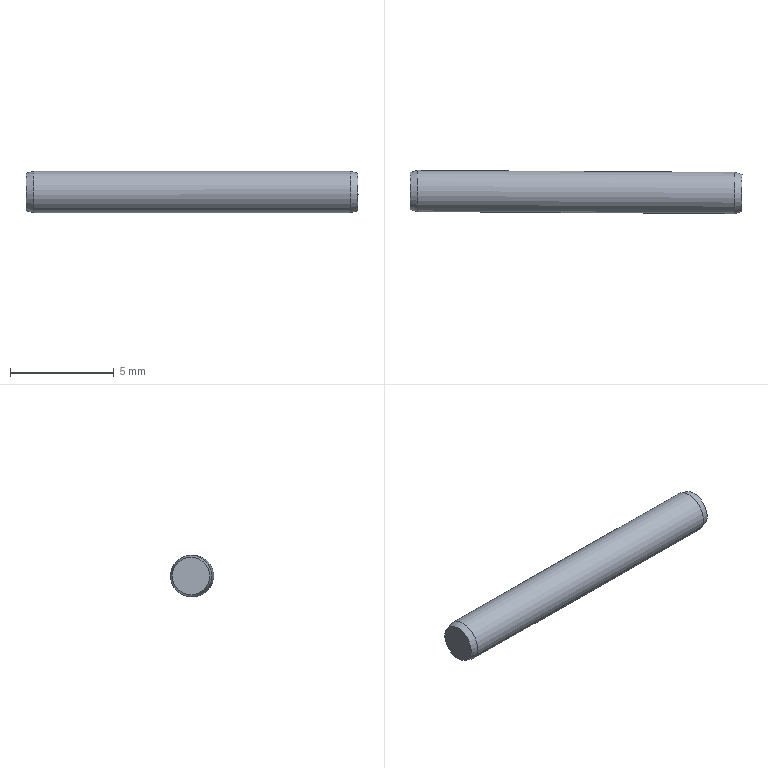Component | NX | GB-T119_1-2000_2X16 | 1 solid | 5 faces | box 16.01 x 2.09 x 2 mm | volume 50 mm3 | plane 2 | cone 2 | cylinder 1 | commonest cylinder face diameters 2 x1
STEP:
#1=CARTESIAN_POINT('',(0.,0.,0.));
#2=DIRECTION('',(0.,0.,1.));
#3=DIRECTION('',(1.,0.,0.));
#4=AXIS2_PLACEMENT_3D('',#1,#2,#3);
#5=CARTESIAN_POINT('',(38.573,-55.252,30.968));
#6=VERTEX_POINT('',#5);
#7=CARTESIAN_POINT('',(38.573,-55.252,30.062));
#8=DIRECTION('',(-1.,0.006117,-0.00004482));
#9=DIRECTION('',(-0.00004482,-0.00000007,1.));
#10=AXIS2_PLACEMENT_3D('',#7,#8,#9);
#11=CIRCLE('',#10,0.9062);
#12=CARTESIAN_POINT('',(38.573,-55.252,30.062));
#13=DIRECTION('',(-1.,0.006117,-0.00004482));
#14=DIRECTION('',(-0.00004482,-0.00000007,1.));
#15=AXIS2_PLACEMENT_3D('',#12,#13,#14);
#16=PLANE('',#15);
#17=CARTESIAN_POINT('',(0.,0.));
#18=DIRECTION('',(1.,-0.));
#19=AXIS2_PLACEMENT_2D('',#17,#18);
#20=CIRCLE('',#19,0.9062);
#21=(GEOMETRIC_REPRESENTATION_CONTEXT(2)PARAMETRIC_REPRESENTATION_CONTEXT()REPRESENTATION_CONTEXT('',''));
#22=DEFINITIONAL_REPRESENTATION('',(#20),#21);
#23=PCURVE('',#16,#22);
#24=CARTESIAN_POINT('',(38.573,-55.252,30.062));
#25=DIRECTION('',(1.,-0.006117,0.00004482));
#26=DIRECTION('',(0.00004482,0.00000007,-1.));
#27=AXIS2_PLACEMENT_3D('',#24,#25,#26);
#28=CONICAL_SURFACE('',#27,0.9062,0.2618);
#29=CARTESIAN_POINT('',(9.425,0.));
#30=DIRECTION('',(-1.,0.));
#31=VECTOR('',#30,1.);
#32=LINE('',#29,#31);
#33=(GEOMETRIC_REPRESENTATION_CONTEXT(2)PARAMETRIC_REPRESENTATION_CONTEXT()REPRESENTATION_CONTEXT('',''));
#34=DEFINITIONAL_REPRESENTATION('',(#32),#33);
#35=PCURVE('',#28,#34);
#36=SURFACE_CURVE('',#11,(#23,#35),.PCURVE_S1.);
#37=EDGE_CURVE('',#6,#6,#36,.T.);
#38=ORIENTED_EDGE('',*,*,#37,.T.);
#39=EDGE_LOOP('',(#38));
#40=FACE_BOUND('',#39,.T.);
#41=ADVANCED_FACE('',(#40),#16,.T.);
#42=CARTESIAN_POINT('',(38.923,-55.254,31.062));
#43=VERTEX_POINT('',#42);
#44=CARTESIAN_POINT('',(38.923,-55.254,30.062));
#45=DIRECTION('',(-1.,0.006117,-0.00004482));
#46=DIRECTION('',(-0.00004482,-0.00000007,1.));
#47=AXIS2_PLACEMENT_3D('',#44,#45,#46);
#48=CIRCLE('',#47,1.);
#49=CARTESIAN_POINT('',(9.425,0.35));
#50=DIRECTION('',(-1.,0.));
#51=VECTOR('',#50,1.);
#52=LINE('',#49,#51);
#53=(GEOMETRIC_REPRESENTATION_CONTEXT(2)PARAMETRIC_REPRESENTATION_CONTEXT()REPRESENTATION_CONTEXT('',''));
#54=DEFINITIONAL_REPRESENTATION('',(#52),#53);
#55=PCURVE('',#28,#54);
#56=CARTESIAN_POINT('',(54.573,-55.35,30.063));
#57=DIRECTION('',(-1.,0.006117,-0.00004482));
#58=DIRECTION('',(-0.00004482,-0.00000007,1.));
#59=AXIS2_PLACEMENT_3D('',#56,#57,#58);
#60=CYLINDRICAL_SURFACE('',#59,1.);
#61=CARTESIAN_POINT('',(0.,15.65));
#62=DIRECTION('',(1.,0.));
#63=VECTOR('',#62,1.);
#64=LINE('',#61,#63);
#65=(GEOMETRIC_REPRESENTATION_CONTEXT(2)PARAMETRIC_REPRESENTATION_CONTEXT()REPRESENTATION_CONTEXT('',''));
#66=DEFINITIONAL_REPRESENTATION('',(#64),#65);
#67=PCURVE('',#60,#66);
#68=SURFACE_CURVE('',#48,(#55,#67),.PCURVE_S1.);
#69=EDGE_CURVE('',#43,#43,#68,.T.);
#70=ORIENTED_EDGE('',*,*,#69,.T.);
#71=CARTESIAN_POINT('',(38.573,-55.252,30.968));
#72=CARTESIAN_POINT('',(38.923,-55.254,31.062));
#73=B_SPLINE_CURVE_WITH_KNOTS('',1,(#71,#72),.UNSPECIFIED.,.F.,.F.,(2,2),(0.,0.3623),.PIECEWISE_BEZIER_KNOTS.);
#74=CARTESIAN_POINT('',(3.142,0.));
#75=DIRECTION('',(0.,1.));
#76=VECTOR('',#75,1.);
#77=LINE('',#74,#76);
#78=(GEOMETRIC_REPRESENTATION_CONTEXT(2)PARAMETRIC_REPRESENTATION_CONTEXT()REPRESENTATION_CONTEXT('',''));
#79=DEFINITIONAL_REPRESENTATION('',(#77),#78);
#80=PCURVE('',#28,#79);
#81=CARTESIAN_POINT('',(9.425,0.));
#82=DIRECTION('',(0.,1.));
#83=VECTOR('',#82,1.);
#84=LINE('',#81,#83);
#85=(GEOMETRIC_REPRESENTATION_CONTEXT(2)PARAMETRIC_REPRESENTATION_CONTEXT()REPRESENTATION_CONTEXT('',''));
#86=DEFINITIONAL_REPRESENTATION('',(#84),#85);
#87=PCURVE('',#28,#86);
#88=SEAM_CURVE('',#73,(#80,#87),.PCURVE_S1.);
#89=EDGE_CURVE('',#6,#43,#88,.T.);
#90=ORIENTED_EDGE('',*,*,#89,.F.);
#91=ORIENTED_EDGE('',*,*,#37,.F.);
#92=ORIENTED_EDGE('',*,*,#89,.T.);
#93=EDGE_LOOP('',(#70,#90,#91,#92));
#94=FACE_BOUND('',#93,.T.);
#95=ADVANCED_FACE('',(#94),#28,.T.);
#96=CARTESIAN_POINT('',(54.223,-55.348,31.063));
#97=VERTEX_POINT('',#96);
#98=CARTESIAN_POINT('',(54.223,-55.348,30.063));
#99=DIRECTION('',(-1.,0.006117,-0.00004482));
#100=DIRECTION('',(-0.00004482,-0.00000007,1.));
#101=AXIS2_PLACEMENT_3D('',#98,#99,#100);
#102=CIRCLE('',#101,1.);
#103=CARTESIAN_POINT('',(0.,0.35));
#104=DIRECTION('',(1.,0.));
#105=VECTOR('',#104,1.);
#106=LINE('',#103,#105);
#107=(GEOMETRIC_REPRESENTATION_CONTEXT(2)PARAMETRIC_REPRESENTATION_CONTEXT()REPRESENTATION_CONTEXT('',''));
#108=DEFINITIONAL_REPRESENTATION('',(#106),#107);
#109=PCURVE('',#60,#108);
#110=CARTESIAN_POINT('',(54.223,-55.348,30.063));
#111=DIRECTION('',(-1.,0.006117,-0.00004482));
#112=DIRECTION('',(-0.00004482,-0.00000007,1.));
#113=AXIS2_PLACEMENT_3D('',#110,#111,#112);
#114=CONICAL_SURFACE('',#113,1.,0.2618);
#115=CARTESIAN_POINT('',(0.,0.));
#116=DIRECTION('',(1.,0.));
#117=VECTOR('',#116,1.);
#118=LINE('',#115,#117);
#119=(GEOMETRIC_REPRESENTATION_CONTEXT(2)PARAMETRIC_REPRESENTATION_CONTEXT()REPRESENTATION_CONTEXT('',''));
#120=DEFINITIONAL_REPRESENTATION('',(#118),#119);
#121=PCURVE('',#114,#120);
#122=SURFACE_CURVE('',#102,(#109,#121),.PCURVE_S1.);
#123=EDGE_CURVE('',#97,#97,#122,.T.);
#124=ORIENTED_EDGE('',*,*,#123,.T.);
#125=CARTESIAN_POINT('',(54.223,-55.348,31.063));
#126=CARTESIAN_POINT('',(38.923,-55.254,31.062));
#127=B_SPLINE_CURVE_WITH_KNOTS('',1,(#125,#126),.UNSPECIFIED.,.F.,.F.,(2,2),(0.35,15.65),.PIECEWISE_BEZIER_KNOTS.);
#128=CARTESIAN_POINT('',(6.283,0.));
#129=DIRECTION('',(0.,1.));
#130=VECTOR('',#129,1.);
#131=LINE('',#128,#130);
#132=(GEOMETRIC_REPRESENTATION_CONTEXT(2)PARAMETRIC_REPRESENTATION_CONTEXT()REPRESENTATION_CONTEXT('',''));
#133=DEFINITIONAL_REPRESENTATION('',(#131),#132);
#134=PCURVE('',#60,#133);
#135=CARTESIAN_POINT('',(0.,0.));
#136=DIRECTION('',(0.,1.));
#137=VECTOR('',#136,1.);
#138=LINE('',#135,#137);
#139=(GEOMETRIC_REPRESENTATION_CONTEXT(2)PARAMETRIC_REPRESENTATION_CONTEXT()REPRESENTATION_CONTEXT('',''));
#140=DEFINITIONAL_REPRESENTATION('',(#138),#139);
#141=PCURVE('',#60,#140);
#142=SEAM_CURVE('',#127,(#134,#141),.PCURVE_S1.);
#143=EDGE_CURVE('',#97,#43,#142,.T.);
#144=ORIENTED_EDGE('',*,*,#143,.T.);
#145=ORIENTED_EDGE('',*,*,#69,.F.);
#146=ORIENTED_EDGE('',*,*,#143,.F.);
#147=EDGE_LOOP('',(#124,#144,#145,#146));
#148=FACE_BOUND('',#147,.T.);
#149=ADVANCED_FACE('',(#148),#60,.T.);
#150=CARTESIAN_POINT('',(54.573,-55.35,30.969));
#151=VERTEX_POINT('',#150);
#152=CARTESIAN_POINT('',(54.573,-55.35,30.063));
#153=DIRECTION('',(-1.,0.006117,-0.00004482));
#154=DIRECTION('',(-0.00004482,-0.00000007,1.));
#155=AXIS2_PLACEMENT_3D('',#152,#153,#154);
#156=CIRCLE('',#155,0.9062);
#157=CARTESIAN_POINT('',(0.,-0.35));
#158=DIRECTION('',(1.,0.));
#159=VECTOR('',#158,1.);
#160=LINE('',#157,#159);
#161=(GEOMETRIC_REPRESENTATION_CONTEXT(2)PARAMETRIC_REPRESENTATION_CONTEXT()REPRESENTATION_CONTEXT('',''));
#162=DEFINITIONAL_REPRESENTATION('',(#160),#161);
#163=PCURVE('',#114,#162);
#164=CARTESIAN_POINT('',(54.573,-55.35,29.157));
#165=DIRECTION('',(1.,-0.006117,0.00004482));
#166=DIRECTION('',(0.00004482,0.00000007,-1.));
#167=AXIS2_PLACEMENT_3D('',#164,#165,#166);
#168=PLANE('',#167);
#169=CARTESIAN_POINT('',(-1.812,0.));
#170=CARTESIAN_POINT('',(-1.812,1.57));
#171=CARTESIAN_POINT('',(-0.4531,0.7848));
#172=CARTESIAN_POINT('',(0.9062,0.));
#173=CARTESIAN_POINT('',(-0.4531,-0.7848));
#174=CARTESIAN_POINT('',(-1.812,-1.57));
#175=CARTESIAN_POINT('',(-1.812,0.));
#176=(BOUNDED_CURVE()B_SPLINE_CURVE(2,(#169,#170,#171,#172,#173,#174,#175),.UNSPECIFIED.,.T.,.F.)B_SPLINE_CURVE_WITH_KNOTS((1,2,2,2,2,1),(-2.094,0.,2.094,4.189,6.283,8.378),.UNSPECIFIED.)CURVE()GEOMETRIC_REPRESENTATION_ITEM()RATIONAL_B_SPLINE_CURVE((1.,0.5,1.,0.5,1.,0.5,1.))REPRESENTATION_ITEM(''));
#177=(GEOMETRIC_REPRESENTATION_CONTEXT(2)PARAMETRIC_REPRESENTATION_CONTEXT()REPRESENTATION_CONTEXT('',''));
#178=DEFINITIONAL_REPRESENTATION('',(#176),#177);
#179=PCURVE('',#168,#178);
#180=SURFACE_CURVE('',#156,(#163,#179),.PCURVE_S1.);
#181=EDGE_CURVE('',#151,#151,#180,.T.);
#182=ORIENTED_EDGE('',*,*,#181,.T.);
#183=CARTESIAN_POINT('',(54.573,-55.35,30.969));
#184=CARTESIAN_POINT('',(54.223,-55.348,31.063));
#185=B_SPLINE_CURVE_WITH_KNOTS('',1,(#183,#184),.UNSPECIFIED.,.F.,.F.,(2,2),(-0.3623,0.),.PIECEWISE_BEZIER_KNOTS.);
#186=CARTESIAN_POINT('',(6.283,0.));
#187=DIRECTION('',(0.,1.));
#188=VECTOR('',#187,1.);
#189=LINE('',#186,#188);
#190=(GEOMETRIC_REPRESENTATION_CONTEXT(2)PARAMETRIC_REPRESENTATION_CONTEXT()REPRESENTATION_CONTEXT('',''));
#191=DEFINITIONAL_REPRESENTATION('',(#189),#190);
#192=PCURVE('',#114,#191);
#193=CARTESIAN_POINT('',(0.,0.));
#194=DIRECTION('',(0.,1.));
#195=VECTOR('',#194,1.);
#196=LINE('',#193,#195);
#197=(GEOMETRIC_REPRESENTATION_CONTEXT(2)PARAMETRIC_REPRESENTATION_CONTEXT()REPRESENTATION_CONTEXT('',''));
#198=DEFINITIONAL_REPRESENTATION('',(#196),#197);
#199=PCURVE('',#114,#198);
#200=SEAM_CURVE('',#185,(#192,#199),.PCURVE_S1.);
#201=EDGE_CURVE('',#151,#97,#200,.T.);
#202=ORIENTED_EDGE('',*,*,#201,.T.);
#203=ORIENTED_EDGE('',*,*,#123,.F.);
#204=ORIENTED_EDGE('',*,*,#201,.F.);
#205=EDGE_LOOP('',(#182,#202,#203,#204));
#206=FACE_BOUND('',#205,.T.);
#207=ADVANCED_FACE('',(#206),#114,.T.);
#208=ORIENTED_EDGE('',*,*,#181,.F.);
#209=EDGE_LOOP('',(#208));
#210=FACE_BOUND('',#209,.T.);
#211=ADVANCED_FACE('',(#210),#168,.T.);
#212=CLOSED_SHELL('',(#41,#95,#149,#207,#211));
#213=MANIFOLD_SOLID_BREP('',#212);
#214=(LENGTH_UNIT()NAMED_UNIT(*)SI_UNIT(.MILLI.,.METRE.));
#215=UNCERTAINTY_MEASURE_WITH_UNIT(LENGTH_MEASURE(0.00001),#214,'','');
#216=(NAMED_UNIT(*)PLANE_ANGLE_UNIT()SI_UNIT($,.RADIAN.));
#217=(NAMED_UNIT(*)SI_UNIT($,.STERADIAN.)SOLID_ANGLE_UNIT());
#218=(GEOMETRIC_REPRESENTATION_CONTEXT(3)GLOBAL_UNCERTAINTY_ASSIGNED_CONTEXT((#215))GLOBAL_UNIT_ASSIGNED_CONTEXT((#214,#216,#217))REPRESENTATION_CONTEXT('',''));
#219=ADVANCED_BREP_SHAPE_REPRESENTATION('',(#4,#213),#218);